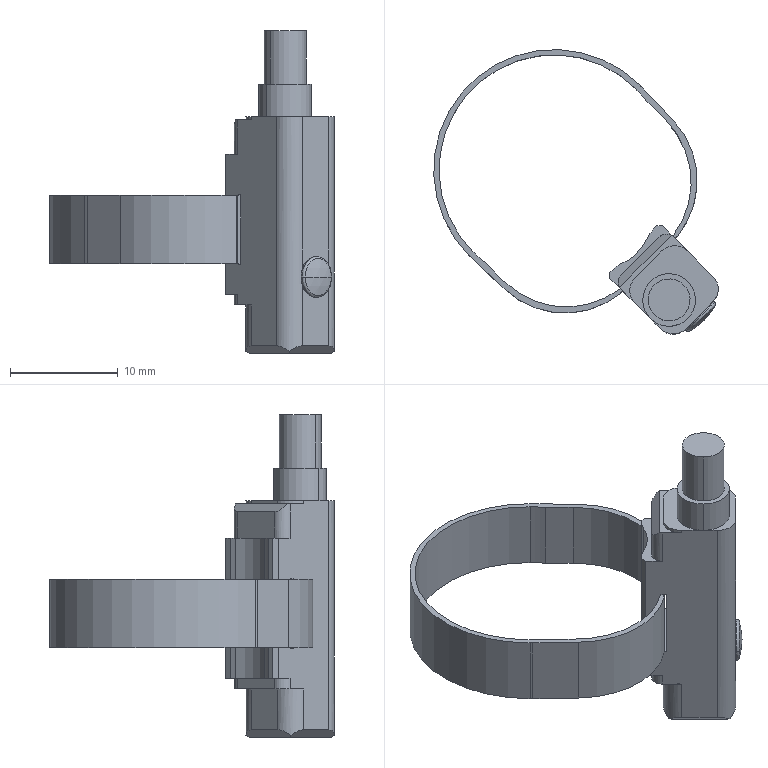Component | SolidWorks | F01AE00111-A2000-21TopEdgeAssembly-1_MA20x250SU(0)+(CS1-M-2)-1_CS1-M-S20-1 | 1 solid | 72 faces | box 26.44 x 26.44 x 30 mm | volume 1490 mm3 | plane 39 | cylinder 29 | sphere 2 | torus 2 | commonest cylinder face diameters 3.4 x6 21.4 x5 16.4 x4 2 x4 22.4 x3 3.8 x2 3.9 x2 4.9 x2
build123d program:
from build123d import *

# Parameters (mm, degrees)
BOSS_EXTRUDE1_DEPTH      = 3.175
BOSS_EXTRUDE1_DEPTH_BACK = 3.175
BOSS_EXTRUDE2_DEPTH      = 18.5
CUT_EXTRUDE1_DEPTH       = 4.5
CUT_EXTRUDE2_DEPTH       = 5.5
CUT_EXTRUDE3_DEPTH       = 18.5
BOSS_EXTRUDE3_DEPTH      = 3.5
CUT_EXTRUDE4_DEPTH       = 3.25
CUT_EXTRUDE4_DEPTH_BACK  = 3.25
SKETCH7_W                = 7.3
SKETCH7_H                = 0.3
SKETCH8_R                = 2.45
BOSS_EXTRUDE4_DEPTH      = 25
SKETCH9_R                = 1.95
BOSS_EXTRUDE5_DEPTH      = 30
BOSS_EXTRUDE6_DEPTH      = 3.2
CUT_EXTRUDE5_DEPTH       = 5
CUT_EXTRUDE5_DEPTH_BACK  = 5
CUT_EXTRUDE6_DEPTH       = 5
CUT_EXTRUDE6_DEPTH_BACK  = 5
CUT_EXTRUDE7_DEPTH       = 10
CUT_EXTRUDE7_DEPTH_BACK  = 10
SKETCH1_R                = 10.7
IR_BANDBORE_D21_4_DEPTH  = 7


with BuildPart() as part:
    # Sketch1_2 → Boss-Extrude1 (new, two sides: drawn at the far end of the back side and taken through both)
    with BuildSketch(Plane(origin=(11.5, 0, 0), x_dir=(0, 0, -1), z_dir=(1, 0, 0)).offset(-BOSS_EXTRUDE1_DEPTH_BACK)):
        with BuildLine():
            Line((11.197, 0.2717), (11.094, 4.499))
            ThreePointArc((11.094, 4.499), (8.624, 10.168), (2.897, 12.5))
            Line((2.897, 12.5), (-2.897, 12.5))
            ThreePointArc((-2.897, 12.5), (-8.624, 10.168), (-11.094, 4.499))
            Line((-11.094, 4.499), (-11.197, 0.2717))
            ThreePointArc((-11.197, 0.2717), (0, -11.2), (11.197, 0.2717))
        make_face()
        with BuildLine():
            Line((-10.6, 4), (-10.6, 0))
            ThreePointArc((-10.6, 0), (0, -10.6), (10.6, 0))
            Line((10.6, 0), (10.6, 4))
            ThreePointArc((10.6, 4), (8.198, 9.798), (2.4, 12.2))
            Line((2.4, 12.2), (-2.4, 12.2))
            ThreePointArc((-2.4, 12.2), (-8.198, 9.798), (-10.6, 4))
        make_face(mode=Mode.SUBTRACT)
    extrude(amount=BOSS_EXTRUDE1_DEPTH + BOSS_EXTRUDE1_DEPTH_BACK)

    # Sketch2 → Boss-Extrude2 (add)
    with BuildSketch(Plane(origin=(0, 0, 0), x_dir=(0, 0, -1), z_dir=(1, 0, 0))):
        with BuildLine():
            Line((-3.45, 10.757), (-3.096, 10.404))
            Line((-3.096, 10.404), (-2.5, 10.404))
            Line((-2.5, 10.404), (-2.5, 10))
            Line((-2.5, 10), (2.5, 10))
            Line((2.5, 10), (2.5, 10.404))
            Line((2.5, 10.404), (3.096, 10.404))
            Line((3.096, 10.404), (3.45, 10.757))
            Line((3.45, 10.757), (3.45, 17.4))
            ThreePointArc((3.45, 17.4), (2.952, 18.602), (1.75, 19.1))
            Line((1.75, 19.1), (-1.75, 19.1))
            ThreePointArc((-1.75, 19.1), (-2.952, 18.602), (-3.45, 17.4))
            Line((-3.45, 17.4), (-3.45, 10.757))
        make_face()
    extrude(amount=BOSS_EXTRUDE2_DEPTH)

    # Sketch3 → Cut-Extrude1 (cut)
    with BuildSketch(Plane(origin=(0, 0, 0), x_dir=(0, 0, -1), z_dir=(1, 0, 0))):
        with BuildLine():
            Line((-3.45, 14.1), (-3.45, 10.757))
            Line((-3.45, 10.757), (-3.096, 10.404))
            Line((-3.096, 10.404), (-2.5, 10.404))
            Line((-2.5, 10.404), (-2.5, 10))
            Line((-2.5, 10), (2.5, 10))
            Line((2.5, 10), (2.5, 10.404))
            Line((2.5, 10.404), (3.096, 10.404))
            Line((3.096, 10.404), (3.45, 10.757))
            Line((3.45, 10.757), (3.45, 14.1))
            ThreePointArc((3.45, 14.1), (2.952, 12.898), (1.75, 12.4))
            Line((1.75, 12.4), (-1.75, 12.4))
            ThreePointArc((-1.75, 12.4), (-2.952, 12.898), (-3.45, 14.1))
        make_face()
    extrude(amount=CUT_EXTRUDE1_DEPTH, mode=Mode.SUBTRACT)

    # Sketch4 → Cut-Extrude2 (cut)
    with BuildSketch(Plane(origin=(0, 0, 0), x_dir=(0, 0, -1), z_dir=(1, 0, 0))):
        with BuildLine():
            Line((-3.45, 12.3), (-3.45, 10.757))
            Line((-3.45, 10.757), (-3.096, 10.404))
            Line((-3.096, 10.404), (-2.5, 10.404))
            Line((-2.5, 10.404), (-2.5, 10))
            Line((-2.5, 10), (2.5, 10))
            Line((2.5, 10), (2.5, 10.404))
            Line((2.5, 10.404), (3.096, 10.404))
            Line((3.096, 10.404), (3.45, 10.757))
            Line((3.45, 10.757), (3.45, 12.3))
            ThreePointArc((3.45, 12.3), (3.157, 11.593), (2.45, 11.3))
            Line((2.45, 11.3), (-2.45, 11.3))
            ThreePointArc((-2.45, 11.3), (-3.157, 11.593), (-3.45, 12.3))
        make_face()
    extrude(amount=CUT_EXTRUDE2_DEPTH, mode=Mode.SUBTRACT)

    # Sketch5 → Cut-Extrude3 (cut)
    with BuildSketch(Plane(origin=(0, 0, 0), x_dir=(0, 0, -1), z_dir=(1, 0, 0))):
        with BuildLine():
            Line((-2.5, 9.6), (2.5, 9.6))
            Line((2.5, 9.6), (2.5, 10.404))
            Line((2.5, 10.404), (2.18, 10.404))
            ThreePointArc((2.18, 10.404), (0, 10.904), (-2.18, 10.404))
            Line((-2.18, 10.404), (-2.5, 10.404))
            Line((-2.5, 10.404), (-2.5, 9.6))
        make_face()
    extrude(amount=CUT_EXTRUDE3_DEPTH, mode=Mode.SUBTRACT)

    # Sketch6 → Boss-Extrude3 (add)
    with BuildSketch(Plane(origin=(18.5, 0, 0), x_dir=(0, 0, -1), z_dir=(1, 0, 0))):
        with BuildLine():
            Line((-1.75, 12.4), (1.75, 12.4))
            ThreePointArc((1.75, 12.4), (2.952, 12.898), (3.45, 14.1))
            Line((3.45, 14.1), (3.45, 17.4))
            ThreePointArc((3.45, 17.4), (2.952, 18.602), (1.75, 19.1))
            Line((1.75, 19.1), (-1.75, 19.1))
            ThreePointArc((-1.75, 19.1), (-2.952, 18.602), (-3.45, 17.4))
            Line((-3.45, 17.4), (-3.45, 14.1))
            ThreePointArc((-3.45, 14.1), (-2.952, 12.898), (-1.75, 12.4))
        make_face()
    extrude(amount=BOSS_EXTRUDE3_DEPTH)

    # Sketch7 → Cut-Extrude4 (cut, two sides: drawn at the far end of the back side and taken through both)
    with BuildSketch(Plane(origin=(11.5, 0, 0), x_dir=(0, 0, -1), z_dir=(1, 0, 0)).offset(-CUT_EXTRUDE4_DEPTH_BACK)):
        with Locations((0, 12.55)):
            Rectangle(SKETCH7_W, SKETCH7_H)
    extrude(amount=CUT_EXTRUDE4_DEPTH + CUT_EXTRUDE4_DEPTH_BACK, mode=Mode.SUBTRACT)

    # Sketch8 → Boss-Extrude4 (add)
    with BuildSketch(Plane(origin=(0, 0, 0), x_dir=(0, 0, -1), z_dir=(1, 0, 0))):
        with Locations((1, 16.1)):
            Circle(SKETCH8_R)
    extrude(amount=BOSS_EXTRUDE4_DEPTH)

    # Sketch9 → Boss-Extrude5 (add)
    with BuildSketch(Plane(origin=(0, 0, 0), x_dir=(0, 0, -1), z_dir=(1, 0, 0))):
        with Locations((1, 16.1)):
            Circle(SKETCH9_R)
    extrude(amount=BOSS_EXTRUDE5_DEPTH)

    # Sketch10 → Boss-Extrude6 (add)
    with BuildSketch(Plane(origin=(18.5, 0, 0), x_dir=(0, 0, -1), z_dir=(1, 0, 0))):
        with BuildLine():
            Line((-2.45, 11.3), (2.45, 11.3))
            ThreePointArc((2.45, 11.3), (3.157, 11.593), (3.45, 12.3))
            Line((3.45, 12.3), (3.45, 14.1))
            ThreePointArc((3.45, 14.1), (2.952, 12.898), (1.75, 12.4))
            Line((1.75, 12.4), (-1.75, 12.4))
            ThreePointArc((-1.75, 12.4), (-2.952, 12.898), (-3.45, 14.1))
            Line((-3.45, 14.1), (-3.45, 12.3))
            ThreePointArc((-3.45, 12.3), (-3.157, 11.593), (-2.45, 11.3))
        make_face()
    extrude(amount=BOSS_EXTRUDE6_DEPTH)

    # Sketch11 → Cut-Extrude5 (cut, two sides: drawn at the far end of the back side and taken through both)
    with BuildSketch(Plane.XY.offset(-CUT_EXTRUDE5_DEPTH_BACK)):
        Polygon((20.993, 11.3), (20.993, 10.3), (22.7, 10.3), (22.7, 12.007), (21.7, 12.007), align=None)
    extrude(amount=CUT_EXTRUDE5_DEPTH + CUT_EXTRUDE5_DEPTH_BACK, mode=Mode.SUBTRACT)

    # Sketch12 → Cut-Extrude6 (cut, two sides: drawn at the far end of the back side and taken through both)
    with BuildSketch(Plane.XY.offset(-CUT_EXTRUDE6_DEPTH_BACK)):
        Polygon((-1, 20.1), (-1, 11.4), (0.7071, 11.4), (0.7071, 12.4), (0, 13.107), (0, 18.393), (0.7071, 19.1), (0.7071, 20.1), align=None)
    extrude(amount=CUT_EXTRUDE6_DEPTH + CUT_EXTRUDE6_DEPTH_BACK, mode=Mode.SUBTRACT)

    # Sketch13 → Cut-Extrude7 (cut, two sides: drawn at the far end of the back side and taken through both)
    with BuildSketch(Plane(origin=(0, 19.1, 0), x_dir=(1, 0, 0), z_dir=(0, 1, 0)).offset(-CUT_EXTRUDE7_DEPTH_BACK)):
        Polygon((-1, -4.45), (0.7071, -4.45), (0.7071, -3.45), (0, -2.743), (0, 2.743), (0.7071, 3.45), (0.7071, 4.45), (-1, 4.45), align=None)
    extrude(amount=CUT_EXTRUDE7_DEPTH + CUT_EXTRUDE7_DEPTH_BACK, mode=Mode.SUBTRACT)

    # Sketch14 → Revolve1 (revolve)
    with BuildSketch(Plane(origin=(7.1, 0, 0), x_dir=(0, 0, -1), z_dir=(1, 0, 0)), mode=Mode.PRIVATE) as revolve1_sk:
        with BuildLine():
            Line((0, 19.1), (-1.9, 19.1))
            Line((-1.9, 19.1), (-1.9, 19.215))
            ThreePointArc((-1.9, 19.215), (-1.85, 19.366), (-1.72, 19.456))
            ThreePointArc((-1.72, 19.456), (-0.8685, 19.639), (0, 19.7))
            Line((0, 19.7), (0, 19.1))
        make_face()
    revolve(revolve1_sk.sketch.rotate(Axis((7.1, 19.7, 0), (0, -1, 0)), 180), axis=Axis((7.1, 19.7, 0), (0, -1, 0)))

    # Sketch1 → IR_BandBore_D21.4 (cut, symmetric)
    with BuildSketch(Plane(origin=(12, 0, 0), x_dir=(0, 0, -1), z_dir=(1, 0, 0))):
        Circle(SKETCH1_R)
    extrude(amount=IR_BANDBORE_D21_4_DEPTH, both=True, mode=Mode.SUBTRACT)


solid = part.part

# Placed as in the assembly
solid = solid.moved(Location((-109.352, 82.548, -314.975), (-90, 45, -90)))